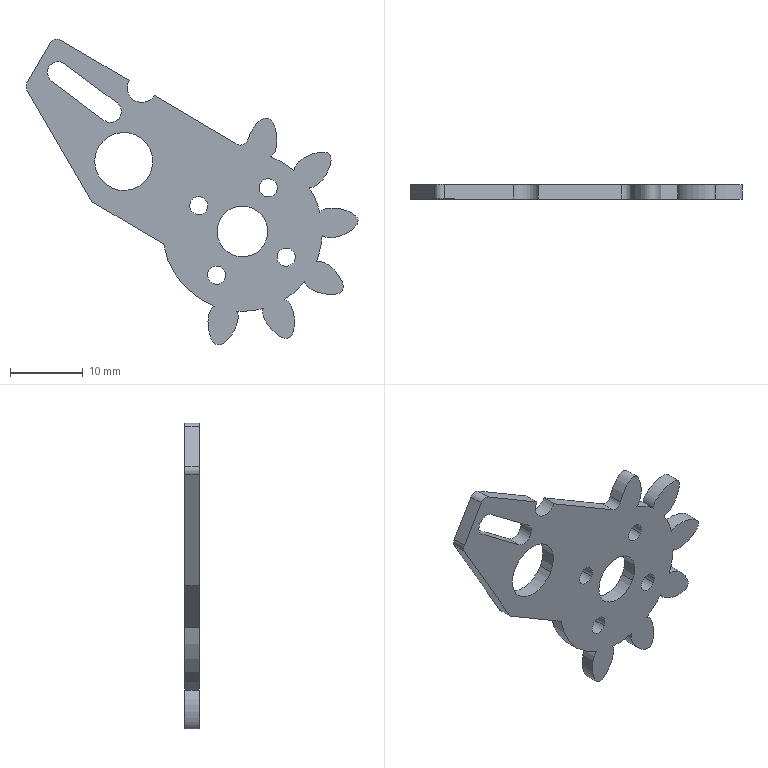Component | SolidWorks | New1-1 | 1 solid | 40 faces | box 45.77 x 2 x 42.16 mm | volume 1414 mm3 | cylinder 25 | plane 9 | spline 6 | commonest cylinder face diameters 2.5 x8 22 x6 3 x3 2 x3 7 x2 8 x2 4 x1
build123d program:
from build123d import *

# Parameters (mm, degrees)
SKETCH1_R           = 3.5
SKETCH1_R_2         = 4
BOSS_EXTRUDE1_DEPTH = 2
FILLET1_R           = 1
FILLET2_R           = 1
FILLET3_R           = 1
SKETCH2_R           = 1.25
CUT_EXTRUDE1_DEPTH  = 10


with BuildPart() as part:
    # Sketch1 → Boss-Extrude1 (new body)
    with BuildSketch(Plane(origin=(0, 0, 0), x_dir=(1, 0, 0), z_dir=(0, 1, 0))):
        with BuildLine():
            Line((5, 0), (0, 0))
            Line((0, 0), (0, -3))
            Line((0, -3), (0, -12))
            ThreePointArc((0, -12), (2, -14), (0, -16))
            Line((0, -16), (0, -17))
            Line((0, -17), (0, -23.51))
            Line((0, -23.51), (0, -30.899))
            add(Edge.make_bspline(
                [(0, -30.899), (-0.3281, -30.504), (-2.23, -29.697), (-7.795, -30.729), (-2.335, -34.908), (-0.8448, -34.159)],
                knots=[0.02571, 0.02571, 0.02571, 0.02571, 0.1753, 0.5, 1, 1, 1, 1], degree=3))
            ThreePointArc((-0.8448, -34.159), (-1, -36), (-0.8448, -37.841))
            add(Edge.make_bspline(
                [(-0.8448, -37.841), (-2.335, -37.092), (-8.956, -42.159), (-0.6214, -42.367), (0.1441, -40.885)],
                knots=[0, 0, 0, 0, 0.5, 1, 1, 1, 1], degree=3))
            ThreePointArc((0.1441, -40.885), (1.101, -42.466), (2.309, -43.864))
            add(Edge.make_bspline(
                [(2.309, -43.864), (0.6628, -44.134), (-1.715, -52.125), (5.149, -47.394), (4.898, -45.745)],
                knots=[0, 0, 0, 0, 0.5, 1, 1, 1, 1], degree=3))
            ThreePointArc((4.898, -45.745), (6.601, -46.462), (8.4, -46.883))
            add(Edge.make_bspline(
                [(8.4, -46.883), (7.227, -48.069), (10, -55.931), (12.773, -48.069), (11.6, -46.883)],
                knots=[0, 0, 0, 0, 0.5, 1, 1, 1, 1], degree=3))
            ThreePointArc((11.6, -46.883), (13.399, -46.462), (15.102, -45.745))
            add(Edge.make_bspline(
                [(15.102, -45.745), (14.851, -47.394), (21.715, -52.125), (19.337, -44.134), (17.691, -43.864)],
                knots=[0, 0, 0, 0, 0.5, 1, 1, 1, 1], degree=3))
            ThreePointArc((17.691, -43.864), (18.899, -42.466), (19.856, -40.885))
            add(Edge.make_bspline(
                [(19.856, -40.885), (20.621, -42.367), (28.956, -42.159), (22.335, -37.092), (20.845, -37.841)],
                knots=[0, 0, 0, 0, 0.5, 1, 1, 1, 1], degree=3))
            ThreePointArc((20.845, -37.841), (20.309, -32.162), (17, -27.515))
            Line((17, -27.515), (17, -21.613))
            Line((17, -21.613), (17, -16))
            Line((17, -16), (8, 0))
            Line((8, 0), (5, 0))
        make_face()
        with Locations(Location((10, -36, 0), (0, 0, 270))):
            Circle(SKETCH1_R, mode=Mode.SUBTRACT)
        with Locations(Location((10, -17, 0), (0, 0, 270))):
            Circle(SKETCH1_R_2, mode=Mode.SUBTRACT)
        with BuildLine():
            ThreePointArc((2.509, -3.167), (3.833, -1.509), (5.491, -2.833))
            Line((5.491, -2.833), (6.491, -11.778))
            ThreePointArc((6.491, -11.778), (5.167, -13.435), (3.509, -12.111))
            Line((3.509, -12.111), (2.509, -3.167))
        make_face(mode=Mode.SUBTRACT)
    extrude(amount=BOSS_EXTRUDE1_DEPTH)

    # Fillet1
    fillet1_edges = [part.edges().sort_by_distance(p)[0] for p in [
        (0, 1, 0),
    ]]
    fillet(fillet1_edges, radius=FILLET1_R)

    # Fillet2
    fillet2_edges = [part.edges().sort_by_distance(p)[0] for p in [
        (8, 1, 0),
    ]]
    fillet(fillet2_edges, radius=FILLET2_R)

    # Fillet3
    fillet3_edges = [part.edges().sort_by_distance(p)[0] for p in [
        (0, 1, 30.899),
    ]]
    fillet(fillet3_edges, radius=FILLET3_R)

    # Sketch2 → Cut-Extrude1 (cut)
    with BuildSketch(Plane(origin=(0, 2, 0), x_dir=(1, 0, 0), z_dir=(0, 1, 0))):
        with Locations(Location((10, -29, 0), (0, 0, 270))):
            Circle(SKETCH2_R)
        with Locations(Location((10, -43, 0), (0, 0, 270))):
            Circle(SKETCH2_R)
        with Locations(Location((17, -36, 0), (0, 0, 270))):
            Circle(SKETCH2_R)
        with Locations(Location((3, -36, 0), (0, 0, 270))):
            Circle(SKETCH2_R)
    extrude(amount=-CUT_EXTRUDE1_DEPTH, mode=Mode.SUBTRACT)


solid = part.part

# Placed as in the assembly
solid = solid.moved(Location((-43.708, 20.649, 80.888), (180, 59.498, -180)))